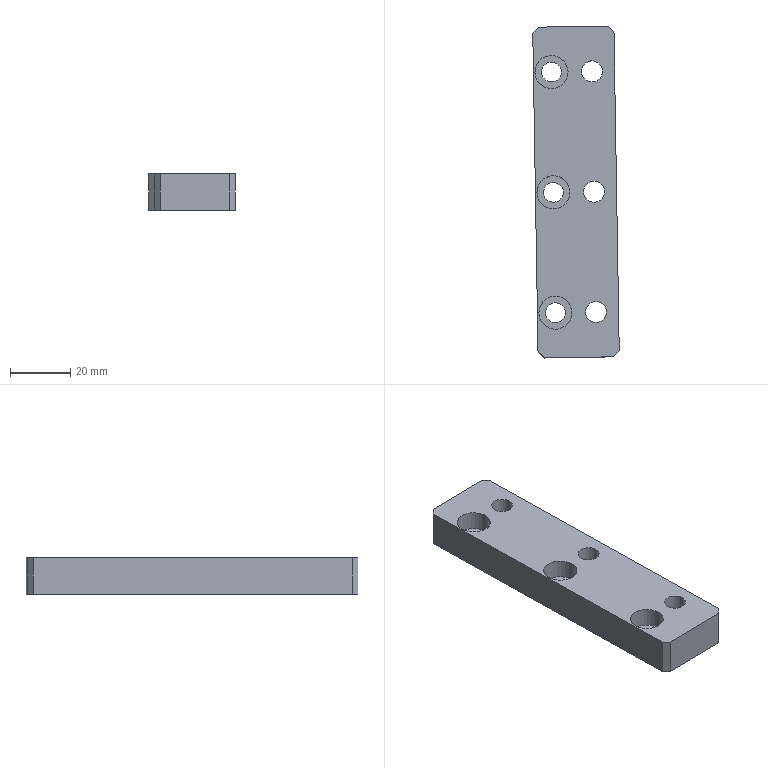Component | SolidWorks | 8TC-A17001-20-09MountingPlate1-2 | 1 solid | 31 faces | box 28.74 x 110.36 x 12 mm | volume 31759 mm3 | cylinder 18 | plane 13 | commonest cylinder face diameters 11 x6 6.6 x6 7 x6 | material A3
build123d program:
from build123d import *

# Parameters (mm, degrees)
SKETCH1_W                                       = 110
SKETCH1_H                                       = 27
BOSS_EXTRUDE1_DEPTH                             = 12
SKETCH2_R                                       = 3.5
CUT_EXTRUDE1_DEPTH                              = 58.89
M6_HEX_SOCKET_HEAD_CAP_SCREW_CBORE1_D           = 6.6
M6_HEX_SOCKET_HEAD_CAP_SCREW_CBORE1_CBORE_D     = 11
M6_HEX_SOCKET_HEAD_CAP_SCREW_CBORE1_CBORE_DEPTH = 6.4
CHAMFER1_SIZE                                   = 2


with BuildPart() as part:
    # Sketch1 → Boss-Extrude1 (new body)
    with BuildSketch(Plane(origin=(0, 0, 0), x_dir=(1, 0, 0), z_dir=(0, 1, 0))):
        Rectangle(SKETCH1_W, SKETCH1_H)
    extrude(amount=BOSS_EXTRUDE1_DEPTH)

    # Sketch2 → Cut-Extrude1 (cut, through all)
    with BuildSketch(Plane(origin=(0, 12, 0), x_dir=(1, 0, 0), z_dir=(0, 1, 0))):
        with Locations(Location((-40, -6, 0), (0, 0, 270))):
            Circle(SKETCH2_R)
        with Locations(Location((0, -6, 0), (0, 0, 270))):
            Circle(SKETCH2_R)
        with Locations(Location((40, -6, 0), (0, 0, 90))):
            Circle(SKETCH2_R)
    extrude(amount=-CUT_EXTRUDE1_DEPTH, mode=Mode.SUBTRACT)

    # M6 Hex Socket Head Cap Screw CBORE1 (through all)
    with Locations(Plane(origin=(0, 0, 0), x_dir=(-1, 0, 0), z_dir=(0, -1, 0))):
        with Locations((40, 7.5), (0, 7.5), (-40, 7.5)):
            CounterBoreHole(M6_HEX_SOCKET_HEAD_CAP_SCREW_CBORE1_D / 2, M6_HEX_SOCKET_HEAD_CAP_SCREW_CBORE1_CBORE_D / 2, M6_HEX_SOCKET_HEAD_CAP_SCREW_CBORE1_CBORE_DEPTH)

    # Chamfer1
    chamfer1_edges = [part.edges().sort_by_distance(p)[0] for p in [
        (55, 6, 13.5),
        (-55, 6, 13.5),
        (-55, 6, -13.5),
        (55, 6, -13.5),
    ]]
    chamfer(chamfer1_edges, length=CHAMFER1_SIZE)


solid = part.part

# Placed as in the assembly
solid = solid.moved(Location((802.019, 201.857, 42.5), (-90, 89.057, 0)))
STEP:
#1=COLOUR_RGB('',0.7922,0.8196,0.9333);
#2=FILL_AREA_STYLE_COLOUR('',#1);
#3=FILL_AREA_STYLE('',(#2));
#4=SURFACE_STYLE_FILL_AREA(#3);
#5=SURFACE_SIDE_STYLE('',(#4));
#6=SURFACE_STYLE_USAGE(.BOTH.,#5);
#7=PRESENTATION_STYLE_ASSIGNMENT((#6));
#8=CARTESIAN_POINT('',(31.471,9.52,1.421));
#9=VERTEX_POINT('',#8);
#10=CARTESIAN_POINT('',(31.038,9.513,1.421));
#11=VERTEX_POINT('',#10);
#12=CARTESIAN_POINT('',(31.254,9.517,1.421));
#13=DIRECTION('',(0.,-0.,1.));
#14=DIRECTION('',(-0.9999,-0.01645,0.));
#15=AXIS2_PLACEMENT_3D('',#12,#13,#14);
#16=CIRCLE('',#15,0.2165);
#17=EDGE_CURVE('',#9,#11,#16,.T.);
#18=ORIENTED_EDGE('',*,*,#17,.F.);
#19=CARTESIAN_POINT('',(31.471,9.52,1.673));
#20=VERTEX_POINT('',#19);
#21=CARTESIAN_POINT('',(31.471,9.52,1.673));
#22=DIRECTION('',(0.,-0.,1.));
#23=VECTOR('',#22,39.37);
#24=LINE('',#21,#23);
#25=EDGE_CURVE('',#9,#20,#24,.T.);
#26=ORIENTED_EDGE('',*,*,#25,.T.);
#27=CARTESIAN_POINT('',(31.038,9.513,1.673));
#28=VERTEX_POINT('',#27);
#29=CARTESIAN_POINT('',(31.254,9.517,1.673));
#30=DIRECTION('',(0.,-0.,1.));
#31=DIRECTION('',(-0.9999,-0.01645,0.));
#32=AXIS2_PLACEMENT_3D('',#29,#30,#31);
#33=CIRCLE('',#32,0.2165);
#34=EDGE_CURVE('',#20,#28,#33,.T.);
#35=ORIENTED_EDGE('',*,*,#34,.T.);
#36=CARTESIAN_POINT('',(31.038,9.513,1.673));
#37=DIRECTION('',(0.,-0.,1.));
#38=VECTOR('',#37,39.37);
#39=LINE('',#36,#38);
#40=EDGE_CURVE('',#11,#28,#39,.T.);
#41=ORIENTED_EDGE('',*,*,#40,.F.);
#42=EDGE_LOOP('',(#18,#26,#35,#41));
#43=FACE_OUTER_BOUND('',#42,.T.);
#44=CARTESIAN_POINT('',(31.254,9.517,1.673));
#45=DIRECTION('',(0.,-0.,1.));
#46=DIRECTION('',(-0.9999,-0.01645,0.));
#47=AXIS2_PLACEMENT_3D('',#44,#45,#46);
#48=CYLINDRICAL_SURFACE('',#47,0.2165);
#49=ADVANCED_FACE('',(#43),#48,.F.);
#50=CARTESIAN_POINT('',(31.384,9.519,1.201));
#51=VERTEX_POINT('',#50);
#52=CARTESIAN_POINT('',(31.125,9.515,1.201));
#53=VERTEX_POINT('',#52);
#54=CARTESIAN_POINT('',(31.254,9.517,1.201));
#55=DIRECTION('',(0.,-0.,1.));
#56=DIRECTION('',(-0.9999,-0.01645,0.));
#57=AXIS2_PLACEMENT_3D('',#54,#55,#56);
#58=CIRCLE('',#57,0.1299);
#59=EDGE_CURVE('',#51,#53,#58,.T.);
#60=ORIENTED_EDGE('',*,*,#59,.F.);
#61=CARTESIAN_POINT('',(31.384,9.519,1.421));
#62=VERTEX_POINT('',#61);
#63=CARTESIAN_POINT('',(31.384,9.519,1.673));
#64=DIRECTION('',(0.,-0.,1.));
#65=VECTOR('',#64,39.37);
#66=LINE('',#63,#65);
#67=EDGE_CURVE('',#51,#62,#66,.T.);
#68=ORIENTED_EDGE('',*,*,#67,.T.);
#69=CARTESIAN_POINT('',(31.125,9.515,1.421));
#70=VERTEX_POINT('',#69);
#71=CARTESIAN_POINT('',(31.254,9.517,1.421));
#72=DIRECTION('',(0.,-0.,1.));
#73=DIRECTION('',(-0.9999,-0.01645,0.));
#74=AXIS2_PLACEMENT_3D('',#71,#72,#73);
#75=CIRCLE('',#74,0.1299);
#76=EDGE_CURVE('',#62,#70,#75,.T.);
#77=ORIENTED_EDGE('',*,*,#76,.T.);
#78=CARTESIAN_POINT('',(31.125,9.515,1.673));
#79=DIRECTION('',(0.,-0.,1.));
#80=VECTOR('',#79,39.37);
#81=LINE('',#78,#80);
#82=EDGE_CURVE('',#53,#70,#81,.T.);
#83=ORIENTED_EDGE('',*,*,#82,.F.);
#84=EDGE_LOOP('',(#60,#68,#77,#83));
#85=FACE_OUTER_BOUND('',#84,.T.);
#86=CARTESIAN_POINT('',(31.254,9.517,1.673));
#87=DIRECTION('',(0.,-0.,1.));
#88=DIRECTION('',(-0.9999,-0.01645,0.));
#89=AXIS2_PLACEMENT_3D('',#86,#87,#88);
#90=CYLINDRICAL_SURFACE('',#89,0.1299);
#91=ADVANCED_FACE('',(#85),#90,.F.);
#92=CARTESIAN_POINT('',(31.497,7.946,1.421));
#93=VERTEX_POINT('',#92);
#94=CARTESIAN_POINT('',(31.064,7.939,1.421));
#95=VERTEX_POINT('',#94);
#96=CARTESIAN_POINT('',(31.28,7.942,1.421));
#97=DIRECTION('',(0.,-0.,1.));
#98=DIRECTION('',(-0.9999,-0.01645,0.));
#99=AXIS2_PLACEMENT_3D('',#96,#97,#98);
#100=CIRCLE('',#99,0.2165);
#101=EDGE_CURVE('',#93,#95,#100,.T.);
#102=ORIENTED_EDGE('',*,*,#101,.F.);
#103=CARTESIAN_POINT('',(31.497,7.946,1.673));
#104=VERTEX_POINT('',#103);
#105=CARTESIAN_POINT('',(31.497,7.946,1.673));
#106=DIRECTION('',(0.,-0.,1.));
#107=VECTOR('',#106,39.37);
#108=LINE('',#105,#107);
#109=EDGE_CURVE('',#93,#104,#108,.T.);
#110=ORIENTED_EDGE('',*,*,#109,.T.);
#111=CARTESIAN_POINT('',(31.064,7.939,1.673));
#112=VERTEX_POINT('',#111);
#113=CARTESIAN_POINT('',(31.28,7.942,1.673));
#114=DIRECTION('',(0.,-0.,1.));
#115=DIRECTION('',(-0.9999,-0.01645,0.));
#116=AXIS2_PLACEMENT_3D('',#113,#114,#115);
#117=CIRCLE('',#116,0.2165);
#118=EDGE_CURVE('',#104,#112,#117,.T.);
#119=ORIENTED_EDGE('',*,*,#118,.T.);
#120=CARTESIAN_POINT('',(31.064,7.939,1.673));
#121=DIRECTION('',(0.,-0.,1.));
#122=VECTOR('',#121,39.37);
#123=LINE('',#120,#122);
#124=EDGE_CURVE('',#95,#112,#123,.T.);
#125=ORIENTED_EDGE('',*,*,#124,.F.);
#126=EDGE_LOOP('',(#102,#110,#119,#125));
#127=FACE_OUTER_BOUND('',#126,.T.);
#128=CARTESIAN_POINT('',(31.28,7.942,1.673));
#129=DIRECTION('',(0.,-0.,1.));
#130=DIRECTION('',(-0.9999,-0.01645,0.));
#131=AXIS2_PLACEMENT_3D('',#128,#129,#130);
#132=CYLINDRICAL_SURFACE('',#131,0.2165);
#133=ADVANCED_FACE('',(#127),#132,.F.);
#134=CARTESIAN_POINT('',(31.41,7.944,1.201));
#135=VERTEX_POINT('',#134);
#136=CARTESIAN_POINT('',(31.15,7.94,1.201));
#137=VERTEX_POINT('',#136);
#138=CARTESIAN_POINT('',(31.28,7.942,1.201));
#139=DIRECTION('',(0.,-0.,1.));
#140=DIRECTION('',(-0.9999,-0.01645,0.));
#141=AXIS2_PLACEMENT_3D('',#138,#139,#140);
#142=CIRCLE('',#141,0.1299);
#143=EDGE_CURVE('',#135,#137,#142,.T.);
#144=ORIENTED_EDGE('',*,*,#143,.F.);
#145=CARTESIAN_POINT('',(31.41,7.944,1.421));
#146=VERTEX_POINT('',#145);
#147=CARTESIAN_POINT('',(31.41,7.944,1.673));
#148=DIRECTION('',(0.,-0.,1.));
#149=VECTOR('',#148,39.37);
#150=LINE('',#147,#149);
#151=EDGE_CURVE('',#135,#146,#150,.T.);
#152=ORIENTED_EDGE('',*,*,#151,.T.);
#153=CARTESIAN_POINT('',(31.15,7.94,1.421));
#154=VERTEX_POINT('',#153);
#155=CARTESIAN_POINT('',(31.28,7.942,1.421));
#156=DIRECTION('',(0.,-0.,1.));
#157=DIRECTION('',(-0.9999,-0.01645,0.));
#158=AXIS2_PLACEMENT_3D('',#155,#156,#157);
#159=CIRCLE('',#158,0.1299);
#160=EDGE_CURVE('',#146,#154,#159,.T.);
#161=ORIENTED_EDGE('',*,*,#160,.T.);
#162=CARTESIAN_POINT('',(31.15,7.94,1.673));
#163=DIRECTION('',(0.,-0.,1.));
#164=VECTOR('',#163,39.37);
#165=LINE('',#162,#164);
#166=EDGE_CURVE('',#137,#154,#165,.T.);
#167=ORIENTED_EDGE('',*,*,#166,.F.);
#168=EDGE_LOOP('',(#144,#152,#161,#167));
#169=FACE_OUTER_BOUND('',#168,.T.);
#170=CARTESIAN_POINT('',(31.28,7.942,1.673));
#171=DIRECTION('',(0.,-0.,1.));
#172=DIRECTION('',(-0.9999,-0.01645,0.));
#173=AXIS2_PLACEMENT_3D('',#170,#171,#172);
#174=CYLINDRICAL_SURFACE('',#173,0.1299);
#175=ADVANCED_FACE('',(#169),#174,.F.);
#176=CARTESIAN_POINT('',(31.523,6.371,1.421));
#177=VERTEX_POINT('',#176);
#178=CARTESIAN_POINT('',(31.09,6.364,1.421));
#179=VERTEX_POINT('',#178);
#180=CARTESIAN_POINT('',(31.306,6.368,1.421));
#181=DIRECTION('',(0.,-0.,1.));
#182=DIRECTION('',(-0.9999,-0.01645,0.));
#183=AXIS2_PLACEMENT_3D('',#180,#181,#182);
#184=CIRCLE('',#183,0.2165);
#185=EDGE_CURVE('',#177,#179,#184,.T.);
#186=ORIENTED_EDGE('',*,*,#185,.F.);
#187=CARTESIAN_POINT('',(31.523,6.371,1.673));
#188=VERTEX_POINT('',#187);
#189=CARTESIAN_POINT('',(31.523,6.371,1.673));
#190=DIRECTION('',(0.,-0.,1.));
#191=VECTOR('',#190,39.37);
#192=LINE('',#189,#191);
#193=EDGE_CURVE('',#177,#188,#192,.T.);
#194=ORIENTED_EDGE('',*,*,#193,.T.);
#195=CARTESIAN_POINT('',(31.09,6.364,1.673));
#196=VERTEX_POINT('',#195);
#197=CARTESIAN_POINT('',(31.306,6.368,1.673));
#198=DIRECTION('',(0.,-0.,1.));
#199=DIRECTION('',(-0.9999,-0.01645,0.));
#200=AXIS2_PLACEMENT_3D('',#197,#198,#199);
#201=CIRCLE('',#200,0.2165);
#202=EDGE_CURVE('',#188,#196,#201,.T.);
#203=ORIENTED_EDGE('',*,*,#202,.T.);
#204=CARTESIAN_POINT('',(31.09,6.364,1.673));
#205=DIRECTION('',(0.,-0.,1.));
#206=VECTOR('',#205,39.37);
#207=LINE('',#204,#206);
#208=EDGE_CURVE('',#179,#196,#207,.T.);
#209=ORIENTED_EDGE('',*,*,#208,.F.);
#210=EDGE_LOOP('',(#186,#194,#203,#209));
#211=FACE_OUTER_BOUND('',#210,.T.);
#212=CARTESIAN_POINT('',(31.306,6.368,1.673));
#213=DIRECTION('',(0.,-0.,1.));
#214=DIRECTION('',(-0.9999,-0.01645,0.));
#215=AXIS2_PLACEMENT_3D('',#212,#213,#214);
#216=CYLINDRICAL_SURFACE('',#215,0.2165);
#217=ADVANCED_FACE('',(#211),#216,.F.);
#218=CARTESIAN_POINT('',(31.436,6.37,1.201));
#219=VERTEX_POINT('',#218);
#220=CARTESIAN_POINT('',(31.176,6.366,1.201));
#221=VERTEX_POINT('',#220);
#222=CARTESIAN_POINT('',(31.306,6.368,1.201));
#223=DIRECTION('',(0.,-0.,1.));
#224=DIRECTION('',(-0.9999,-0.01645,0.));
#225=AXIS2_PLACEMENT_3D('',#222,#223,#224);
#226=CIRCLE('',#225,0.1299);
#227=EDGE_CURVE('',#219,#221,#226,.T.);
#228=ORIENTED_EDGE('',*,*,#227,.F.);
#229=CARTESIAN_POINT('',(31.436,6.37,1.421));
#230=VERTEX_POINT('',#229);
#231=CARTESIAN_POINT('',(31.436,6.37,1.673));
#232=DIRECTION('',(0.,-0.,1.));
#233=VECTOR('',#232,39.37);
#234=LINE('',#231,#233);
#235=EDGE_CURVE('',#219,#230,#234,.T.);
#236=ORIENTED_EDGE('',*,*,#235,.T.);
#237=CARTESIAN_POINT('',(31.176,6.366,1.421));
#238=VERTEX_POINT('',#237);
#239=CARTESIAN_POINT('',(31.306,6.368,1.421));
#240=DIRECTION('',(0.,-0.,1.));
#241=DIRECTION('',(-0.9999,-0.01645,0.));
#242=AXIS2_PLACEMENT_3D('',#239,#240,#241);
#243=CIRCLE('',#242,0.1299);
#244=EDGE_CURVE('',#230,#238,#243,.T.);
#245=ORIENTED_EDGE('',*,*,#244,.T.);
#246=CARTESIAN_POINT('',(31.176,6.366,1.673));
#247=DIRECTION('',(0.,-0.,1.));
#248=VECTOR('',#247,39.37);
#249=LINE('',#246,#248);
#250=EDGE_CURVE('',#221,#238,#249,.T.);
#251=ORIENTED_EDGE('',*,*,#250,.F.);
#252=EDGE_LOOP('',(#228,#236,#245,#251));
#253=FACE_OUTER_BOUND('',#252,.T.);
#254=CARTESIAN_POINT('',(31.306,6.368,1.673));
#255=DIRECTION('',(0.,-0.,1.));
#256=DIRECTION('',(-0.9999,-0.01645,0.));
#257=AXIS2_PLACEMENT_3D('',#254,#255,#256);
#258=CYLINDRICAL_SURFACE('',#257,0.1299);
#259=ADVANCED_FACE('',(#253),#258,.F.);
#260=CARTESIAN_POINT('',(31.7,6.374,1.673));
#261=VERTEX_POINT('',#260);
#262=CARTESIAN_POINT('',(31.975,6.379,1.673));
#263=VERTEX_POINT('',#262);
#264=CARTESIAN_POINT('',(31.838,6.376,1.673));
#265=DIRECTION('',(-0.,0.,-1.));
#266=DIRECTION('',(-0.9999,-0.01645,0.));
#267=AXIS2_PLACEMENT_3D('',#264,#265,#266);
#268=CIRCLE('',#267,0.1378);
#269=EDGE_CURVE('',#261,#263,#268,.T.);
#270=ORIENTED_EDGE('',*,*,#269,.F.);
#271=CARTESIAN_POINT('',(31.7,6.374,1.201));
#272=VERTEX_POINT('',#271);
#273=CARTESIAN_POINT('',(31.7,6.374,1.673));
#274=DIRECTION('',(-0.,0.,-1.));
#275=VECTOR('',#274,39.37);
#276=LINE('',#273,#275);
#277=EDGE_CURVE('',#261,#272,#276,.T.);
#278=ORIENTED_EDGE('',*,*,#277,.T.);
#279=CARTESIAN_POINT('',(31.975,6.379,1.201));
#280=VERTEX_POINT('',#279);
#281=CARTESIAN_POINT('',(31.838,6.376,1.201));
#282=DIRECTION('',(-0.,0.,-1.));
#283=DIRECTION('',(-0.9999,-0.01645,0.));
#284=AXIS2_PLACEMENT_3D('',#281,#282,#283);
#285=CIRCLE('',#284,0.1378);
#286=EDGE_CURVE('',#272,#280,#285,.T.);
#287=ORIENTED_EDGE('',*,*,#286,.T.);
#288=CARTESIAN_POINT('',(31.975,6.379,1.673));
#289=DIRECTION('',(-0.,0.,-1.));
#290=VECTOR('',#289,39.37);
#291=LINE('',#288,#290);
#292=EDGE_CURVE('',#263,#280,#291,.T.);
#293=ORIENTED_EDGE('',*,*,#292,.F.);
#294=EDGE_LOOP('',(#270,#278,#287,#293));
#295=FACE_OUTER_BOUND('',#294,.T.);
#296=CARTESIAN_POINT('',(31.838,6.376,1.673));
#297=DIRECTION('',(-0.,0.,-1.));
#298=DIRECTION('',(0.9999,0.01645,0.));
#299=AXIS2_PLACEMENT_3D('',#296,#297,#298);
#300=CYLINDRICAL_SURFACE('',#299,0.1378);
#301=ADVANCED_FACE('',(#295),#300,.F.);
#302=CARTESIAN_POINT('',(31.674,7.949,1.673));
#303=VERTEX_POINT('',#302);
#304=CARTESIAN_POINT('',(31.95,7.953,1.673));
#305=VERTEX_POINT('',#304);
#306=CARTESIAN_POINT('',(31.812,7.951,1.673));
#307=DIRECTION('',(-0.,0.,-1.));
#308=DIRECTION('',(0.9999,0.01645,0.));
#309=AXIS2_PLACEMENT_3D('',#306,#307,#308);
#310=CIRCLE('',#309,0.1378);
#311=EDGE_CURVE('',#303,#305,#310,.T.);
#312=ORIENTED_EDGE('',*,*,#311,.F.);
#313=CARTESIAN_POINT('',(31.674,7.949,1.201));
#314=VERTEX_POINT('',#313);
#315=CARTESIAN_POINT('',(31.674,7.949,1.673));
#316=DIRECTION('',(-0.,0.,-1.));
#317=VECTOR('',#316,39.37);
#318=LINE('',#315,#317);
#319=EDGE_CURVE('',#303,#314,#318,.T.);
#320=ORIENTED_EDGE('',*,*,#319,.T.);
#321=CARTESIAN_POINT('',(31.95,7.953,1.201));
#322=VERTEX_POINT('',#321);
#323=CARTESIAN_POINT('',(31.812,7.951,1.201));
#324=DIRECTION('',(-0.,0.,-1.));
#325=DIRECTION('',(0.9999,0.01645,0.));
#326=AXIS2_PLACEMENT_3D('',#323,#324,#325);
#327=CIRCLE('',#326,0.1378);
#328=EDGE_CURVE('',#314,#322,#327,.T.);
#329=ORIENTED_EDGE('',*,*,#328,.T.);
#330=CARTESIAN_POINT('',(31.95,7.953,1.673));
#331=DIRECTION('',(-0.,0.,-1.));
#332=VECTOR('',#331,39.37);
#333=LINE('',#330,#332);
#334=EDGE_CURVE('',#305,#322,#333,.T.);
#335=ORIENTED_EDGE('',*,*,#334,.F.);
#336=EDGE_LOOP('',(#312,#320,#329,#335));
#337=FACE_OUTER_BOUND('',#336,.T.);
#338=CARTESIAN_POINT('',(31.812,7.951,1.673));
#339=DIRECTION('',(-0.,0.,-1.));
#340=DIRECTION('',(0.9999,0.01645,0.));
#341=AXIS2_PLACEMENT_3D('',#338,#339,#340);
#342=CYLINDRICAL_SURFACE('',#341,0.1378);
#343=ADVANCED_FACE('',(#337),#342,.F.);
#344=CARTESIAN_POINT('',(31.648,9.523,1.673));
#345=VERTEX_POINT('',#344);
#346=CARTESIAN_POINT('',(31.924,9.528,1.673));
#347=VERTEX_POINT('',#346);
#348=CARTESIAN_POINT('',(31.786,9.526,1.673));
#349=DIRECTION('',(-0.,0.,-1.));
#350=DIRECTION('',(0.9999,0.01645,0.));
#351=AXIS2_PLACEMENT_3D('',#348,#349,#350);
#352=CIRCLE('',#351,0.1378);
#353=EDGE_CURVE('',#345,#347,#352,.T.);
#354=ORIENTED_EDGE('',*,*,#353,.F.);
#355=CARTESIAN_POINT('',(31.648,9.523,1.201));
#356=VERTEX_POINT('',#355);
#357=CARTESIAN_POINT('',(31.648,9.523,1.673));
#358=DIRECTION('',(-0.,0.,-1.));
#359=VECTOR('',#358,39.37);
#360=LINE('',#357,#359);
#361=EDGE_CURVE('',#345,#356,#360,.T.);
#362=ORIENTED_EDGE('',*,*,#361,.T.);
#363=CARTESIAN_POINT('',(31.924,9.528,1.201));
#364=VERTEX_POINT('',#363);
#365=CARTESIAN_POINT('',(31.786,9.526,1.201));
#366=DIRECTION('',(-0.,0.,-1.));
#367=DIRECTION('',(0.9999,0.01645,0.));
#368=AXIS2_PLACEMENT_3D('',#365,#366,#367);
#369=CIRCLE('',#368,0.1378);
#370=EDGE_CURVE('',#356,#364,#369,.T.);
#371=ORIENTED_EDGE('',*,*,#370,.T.);
#372=CARTESIAN_POINT('',(31.924,9.528,1.673));
#373=DIRECTION('',(-0.,0.,-1.));
#374=VECTOR('',#373,39.37);
#375=LINE('',#372,#374);
#376=EDGE_CURVE('',#347,#364,#375,.T.);
#377=ORIENTED_EDGE('',*,*,#376,.F.);
#378=EDGE_LOOP('',(#354,#362,#371,#377));
#379=FACE_OUTER_BOUND('',#378,.T.);
#380=CARTESIAN_POINT('',(31.786,9.526,1.673));
#381=DIRECTION('',(-0.,0.,-1.));
#382=DIRECTION('',(0.9999,0.01645,0.));
#383=AXIS2_PLACEMENT_3D('',#380,#381,#382);
#384=CYLINDRICAL_SURFACE('',#383,0.1378);
#385=ADVANCED_FACE('',(#379),#384,.F.);
#386=CARTESIAN_POINT('',(32.064,5.79,1.673));
#387=VERTEX_POINT('',#386);
#388=CARTESIAN_POINT('',(31.158,5.775,1.673));
#389=VERTEX_POINT('',#388);
#390=CARTESIAN_POINT('',(31.08,5.773,1.673));
#391=DIRECTION('',(-0.9999,-0.01645,0.));
#392=VECTOR('',#391,39.37);
#393=LINE('',#390,#392);
#394=EDGE_CURVE('',#387,#389,#393,.T.);
#395=ORIENTED_EDGE('',*,*,#394,.T.);
#396=CARTESIAN_POINT('',(31.158,5.775,1.201));
#397=VERTEX_POINT('',#396);
#398=CARTESIAN_POINT('',(31.158,5.775,1.201));
#399=DIRECTION('',(-0.,0.,-1.));
#400=VECTOR('',#399,39.37);
#401=LINE('',#398,#400);
#402=EDGE_CURVE('',#389,#397,#401,.T.);
#403=ORIENTED_EDGE('',*,*,#402,.T.);
#404=CARTESIAN_POINT('',(32.064,5.79,1.201));
#405=VERTEX_POINT('',#404);
#406=CARTESIAN_POINT('',(31.08,5.773,1.201));
#407=DIRECTION('',(-0.9999,-0.01645,0.));
#408=VECTOR('',#407,39.37);
#409=LINE('',#406,#408);
#410=EDGE_CURVE('',#405,#397,#409,.T.);
#411=ORIENTED_EDGE('',*,*,#410,.F.);
#412=CARTESIAN_POINT('',(32.064,5.79,1.201));
#413=DIRECTION('',(0.,-0.,1.));
#414=VECTOR('',#413,39.37);
#415=LINE('',#412,#414);
#416=EDGE_CURVE('',#405,#387,#415,.T.);
#417=ORIENTED_EDGE('',*,*,#416,.T.);
#418=EDGE_LOOP('',(#395,#403,#411,#417));
#419=FACE_OUTER_BOUND('',#418,.T.);
#420=CARTESIAN_POINT('',(31.08,5.773,1.201));
#421=DIRECTION('',(-0.01645,0.9999,0.));
#422=DIRECTION('',(0.9999,0.01645,-0.));
#423=AXIS2_PLACEMENT_3D('',#420,#421,#422);
#424=PLANE('',#423);
#425=ADVANCED_FACE('',(#419),#424,.F.);
#426=CARTESIAN_POINT('',(31.078,5.852,1.673));
#427=VERTEX_POINT('',#426);
#428=CARTESIAN_POINT('',(31.01,10.025,1.673));
#429=VERTEX_POINT('',#428);
#430=CARTESIAN_POINT('',(31.009,10.103,1.673));
#431=DIRECTION('',(-0.01645,0.9999,0.));
#432=VECTOR('',#431,39.37);
#433=LINE('',#430,#432);
#434=EDGE_CURVE('',#427,#429,#433,.T.);
#435=ORIENTED_EDGE('',*,*,#434,.T.);
#436=CARTESIAN_POINT('',(31.01,10.025,1.201));
#437=VERTEX_POINT('',#436);
#438=CARTESIAN_POINT('',(31.01,10.025,1.201));
#439=DIRECTION('',(-0.,0.,-1.));
#440=VECTOR('',#439,39.37);
#441=LINE('',#438,#440);
#442=EDGE_CURVE('',#429,#437,#441,.T.);
#443=ORIENTED_EDGE('',*,*,#442,.T.);
#444=CARTESIAN_POINT('',(31.078,5.852,1.201));
#445=VERTEX_POINT('',#444);
#446=CARTESIAN_POINT('',(31.009,10.103,1.201));
#447=DIRECTION('',(-0.01645,0.9999,0.));
#448=VECTOR('',#447,39.37);
#449=LINE('',#446,#448);
#450=EDGE_CURVE('',#445,#437,#449,.T.);
#451=ORIENTED_EDGE('',*,*,#450,.F.);
#452=CARTESIAN_POINT('',(31.078,5.852,1.201));
#453=DIRECTION('',(0.,-0.,1.));
#454=VECTOR('',#453,39.37);
#455=LINE('',#452,#454);
#456=EDGE_CURVE('',#445,#427,#455,.T.);
#457=ORIENTED_EDGE('',*,*,#456,.T.);
#458=EDGE_LOOP('',(#435,#443,#451,#457));
#459=FACE_OUTER_BOUND('',#458,.T.);
#460=CARTESIAN_POINT('',(31.009,10.103,1.201));
#461=DIRECTION('',(0.9999,0.01645,-0.));
#462=DIRECTION('',(0.01645,-0.9999,-0.));
#463=AXIS2_PLACEMENT_3D('',#460,#461,#462);
#464=PLANE('',#463);
#465=ADVANCED_FACE('',(#459),#464,.F.);
#466=CARTESIAN_POINT('',(31.087,10.105,1.201));
#467=VERTEX_POINT('',#466);
#468=CARTESIAN_POINT('',(31.993,10.12,1.201));
#469=VERTEX_POINT('',#468);
#470=CARTESIAN_POINT('',(31.009,10.103,1.201));
#471=DIRECTION('',(0.9999,0.01645,-0.));
#472=VECTOR('',#471,39.37);
#473=LINE('',#470,#472);
#474=EDGE_CURVE('',#467,#469,#473,.T.);
#475=ORIENTED_EDGE('',*,*,#474,.F.);
#476=CARTESIAN_POINT('',(31.087,10.105,1.673));
#477=VERTEX_POINT('',#476);
#478=CARTESIAN_POINT('',(31.087,10.105,1.201));
#479=DIRECTION('',(0.,-0.,1.));
#480=VECTOR('',#479,39.37);
#481=LINE('',#478,#480);
#482=EDGE_CURVE('',#467,#477,#481,.T.);
#483=ORIENTED_EDGE('',*,*,#482,.T.);
#484=CARTESIAN_POINT('',(31.993,10.12,1.673));
#485=VERTEX_POINT('',#484);
#486=CARTESIAN_POINT('',(31.009,10.103,1.673));
#487=DIRECTION('',(0.9999,0.01645,-0.));
#488=VECTOR('',#487,39.37);
#489=LINE('',#486,#488);
#490=EDGE_CURVE('',#477,#485,#489,.T.);
#491=ORIENTED_EDGE('',*,*,#490,.T.);
#492=CARTESIAN_POINT('',(31.993,10.12,1.201));
#493=DIRECTION('',(-0.,0.,-1.));
#494=VECTOR('',#493,39.37);
#495=LINE('',#492,#494);
#496=EDGE_CURVE('',#485,#469,#495,.T.);
#497=ORIENTED_EDGE('',*,*,#496,.T.);
#498=EDGE_LOOP('',(#475,#483,#491,#497));
#499=FACE_OUTER_BOUND('',#498,.T.);
#500=CARTESIAN_POINT('',(31.009,10.103,1.201));
#501=DIRECTION('',(0.01645,-0.9999,-0.));
#502=DIRECTION('',(-0.9999,-0.01645,0.));
#503=AXIS2_PLACEMENT_3D('',#500,#501,#502);
#504=PLANE('',#503);
#505=ADVANCED_FACE('',(#499),#504,.F.);
#506=CARTESIAN_POINT('',(32.073,10.042,1.673));
#507=VERTEX_POINT('',#506);
#508=CARTESIAN_POINT('',(32.141,5.87,1.673));
#509=VERTEX_POINT('',#508);
#510=CARTESIAN_POINT('',(32.071,10.121,1.673));
#511=DIRECTION('',(0.01645,-0.9999,-0.));
#512=VECTOR('',#511,39.37);
#513=LINE('',#510,#512);
#514=EDGE_CURVE('',#507,#509,#513,.T.);
#515=ORIENTED_EDGE('',*,*,#514,.T.);
#516=CARTESIAN_POINT('',(32.141,5.87,1.201));
#517=VERTEX_POINT('',#516);
#518=CARTESIAN_POINT('',(32.141,5.87,1.201));
#519=DIRECTION('',(-0.,0.,-1.));
#520=VECTOR('',#519,39.37);
#521=LINE('',#518,#520);
#522=EDGE_CURVE('',#509,#517,#521,.T.);
#523=ORIENTED_EDGE('',*,*,#522,.T.);
#524=CARTESIAN_POINT('',(32.073,10.042,1.201));
#525=VERTEX_POINT('',#524);
#526=CARTESIAN_POINT('',(32.071,10.121,1.201));
#527=DIRECTION('',(0.01645,-0.9999,-0.));
#528=VECTOR('',#527,39.37);
#529=LINE('',#526,#528);
#530=EDGE_CURVE('',#525,#517,#529,.T.);
#531=ORIENTED_EDGE('',*,*,#530,.F.);
#532=CARTESIAN_POINT('',(32.073,10.042,1.201));
#533=DIRECTION('',(0.,-0.,1.));
#534=VECTOR('',#533,39.37);
#535=LINE('',#532,#534);
#536=EDGE_CURVE('',#525,#507,#535,.T.);
#537=ORIENTED_EDGE('',*,*,#536,.T.);
#538=EDGE_LOOP('',(#515,#523,#531,#537));
#539=FACE_OUTER_BOUND('',#538,.T.);
#540=CARTESIAN_POINT('',(32.071,10.121,1.201));
#541=DIRECTION('',(-0.9999,-0.01645,0.));
#542=DIRECTION('',(-0.01645,0.9999,0.));
#543=AXIS2_PLACEMENT_3D('',#540,#541,#542);
#544=PLANE('',#543);
#545=ADVANCED_FACE('',(#539),#544,.F.);
#546=CARTESIAN_POINT('',(31.254,9.517,1.201));
#547=DIRECTION('',(0.,-0.,1.));
#548=DIRECTION('',(-0.9999,-0.01645,0.));
#549=AXIS2_PLACEMENT_3D('',#546,#547,#548);
#550=CIRCLE('',#549,0.1299);
#551=EDGE_CURVE('',#53,#51,#550,.T.);
#552=ORIENTED_EDGE('',*,*,#551,.T.);
#553=ORIENTED_EDGE('',*,*,#59,.T.);
#554=EDGE_LOOP('',(#552,#553));
#555=FACE_BOUND('',#554,.T.);
#556=CARTESIAN_POINT('',(31.28,7.942,1.201));
#557=DIRECTION('',(0.,-0.,1.));
#558=DIRECTION('',(-0.9999,-0.01645,0.));
#559=AXIS2_PLACEMENT_3D('',#556,#557,#558);
#560=CIRCLE('',#559,0.1299);
#561=EDGE_CURVE('',#137,#135,#560,.T.);
#562=ORIENTED_EDGE('',*,*,#561,.T.);
#563=ORIENTED_EDGE('',*,*,#143,.T.);
#564=EDGE_LOOP('',(#562,#563));
#565=FACE_BOUND('',#564,.T.);
#566=CARTESIAN_POINT('',(31.306,6.368,1.201));
#567=DIRECTION('',(0.,-0.,1.));
#568=DIRECTION('',(-0.9999,-0.01645,0.));
#569=AXIS2_PLACEMENT_3D('',#566,#567,#568);
#570=CIRCLE('',#569,0.1299);
#571=EDGE_CURVE('',#221,#219,#570,.T.);
#572=ORIENTED_EDGE('',*,*,#571,.T.);
#573=ORIENTED_EDGE('',*,*,#227,.T.);
#574=EDGE_LOOP('',(#572,#573));
#575=FACE_BOUND('',#574,.T.);
#576=CARTESIAN_POINT('',(31.838,6.376,1.201));
#577=DIRECTION('',(-0.,0.,-1.));
#578=DIRECTION('',(-0.9999,-0.01645,0.));
#579=AXIS2_PLACEMENT_3D('',#576,#577,#578);
#580=CIRCLE('',#579,0.1378);
#581=EDGE_CURVE('',#280,#272,#580,.T.);
#582=ORIENTED_EDGE('',*,*,#581,.F.);
#583=ORIENTED_EDGE('',*,*,#286,.F.);
#584=EDGE_LOOP('',(#582,#583));
#585=FACE_BOUND('',#584,.T.);
#586=CARTESIAN_POINT('',(31.812,7.951,1.201));
#587=DIRECTION('',(-0.,0.,-1.));
#588=DIRECTION('',(0.9999,0.01645,0.));
#589=AXIS2_PLACEMENT_3D('',#586,#587,#588);
#590=CIRCLE('',#589,0.1378);
#591=EDGE_CURVE('',#322,#314,#590,.T.);
#592=ORIENTED_EDGE('',*,*,#591,.F.);
#593=ORIENTED_EDGE('',*,*,#328,.F.);
#594=EDGE_LOOP('',(#592,#593));
#595=FACE_BOUND('',#594,.T.);
#596=CARTESIAN_POINT('',(31.786,9.526,1.201));
#597=DIRECTION('',(-0.,0.,-1.));
#598=DIRECTION('',(0.9999,0.01645,0.));
#599=AXIS2_PLACEMENT_3D('',#596,#597,#598);
#600=CIRCLE('',#599,0.1378);
#601=EDGE_CURVE('',#364,#356,#600,.T.);
#602=ORIENTED_EDGE('',*,*,#601,.F.);
#603=ORIENTED_EDGE('',*,*,#370,.F.);
#604=EDGE_LOOP('',(#602,#603));
#605=FACE_BOUND('',#604,.T.);
#606=ORIENTED_EDGE('',*,*,#450,.T.);
#607=CARTESIAN_POINT('',(30.245,9.234,1.201));
#608=DIRECTION('',(0.6954,0.7186,-0.));
#609=VECTOR('',#608,39.37);
#610=LINE('',#607,#609);
#611=EDGE_CURVE('',#437,#467,#610,.T.);
#612=ORIENTED_EDGE('',*,*,#611,.T.);
#613=ORIENTED_EDGE('',*,*,#474,.T.);
#614=CARTESIAN_POINT('',(32.863,9.278,1.201));
#615=DIRECTION('',(0.7186,-0.6954,-0.));
#616=VECTOR('',#615,39.37);
#617=LINE('',#614,#616);
#618=EDGE_CURVE('',#469,#525,#617,.T.);
#619=ORIENTED_EDGE('',*,*,#618,.T.);
#620=ORIENTED_EDGE('',*,*,#530,.T.);
#621=CARTESIAN_POINT('',(32.906,6.66,1.201));
#622=DIRECTION('',(-0.6954,-0.7186,0.));
#623=VECTOR('',#622,39.37);
#624=LINE('',#621,#623);
#625=EDGE_CURVE('',#517,#405,#624,.T.);
#626=ORIENTED_EDGE('',*,*,#625,.T.);
#627=ORIENTED_EDGE('',*,*,#410,.T.);
#628=CARTESIAN_POINT('',(30.288,6.617,1.201));
#629=DIRECTION('',(-0.7186,0.6954,0.));
#630=VECTOR('',#629,39.37);
#631=LINE('',#628,#630);
#632=EDGE_CURVE('',#397,#445,#631,.T.);
#633=ORIENTED_EDGE('',*,*,#632,.T.);
#634=EDGE_LOOP('',(#606,#612,#613,#619,#620,#626,#627,#633));
#635=FACE_OUTER_BOUND('',#634,.T.);
#636=CARTESIAN_POINT('',(31.576,7.947,1.201));
#637=DIRECTION('',(-0.,0.,-1.));
#638=DIRECTION('',(0.9999,0.01645,-0.));
#639=AXIS2_PLACEMENT_3D('',#636,#637,#638);
#640=PLANE('',#639);
#641=ADVANCED_FACE('',(#555,#565,#575,#585,#595,#605,#635),#640,.T.);
#642=CARTESIAN_POINT('',(31.254,9.517,1.673));
#643=DIRECTION('',(0.,-0.,1.));
#644=DIRECTION('',(-0.9999,-0.01645,0.));
#645=AXIS2_PLACEMENT_3D('',#642,#643,#644);
#646=CIRCLE('',#645,0.2165);
#647=EDGE_CURVE('',#28,#20,#646,.T.);
#648=ORIENTED_EDGE('',*,*,#647,.F.);
#649=ORIENTED_EDGE('',*,*,#34,.F.);
#650=EDGE_LOOP('',(#648,#649));
#651=FACE_BOUND('',#650,.T.);
#652=CARTESIAN_POINT('',(31.28,7.942,1.673));
#653=DIRECTION('',(0.,-0.,1.));
#654=DIRECTION('',(-0.9999,-0.01645,0.));
#655=AXIS2_PLACEMENT_3D('',#652,#653,#654);
#656=CIRCLE('',#655,0.2165);
#657=EDGE_CURVE('',#112,#104,#656,.T.);
#658=ORIENTED_EDGE('',*,*,#657,.F.);
#659=ORIENTED_EDGE('',*,*,#118,.F.);
#660=EDGE_LOOP('',(#658,#659));
#661=FACE_BOUND('',#660,.T.);
#662=CARTESIAN_POINT('',(31.306,6.368,1.673));
#663=DIRECTION('',(0.,-0.,1.));
#664=DIRECTION('',(-0.9999,-0.01645,0.));
#665=AXIS2_PLACEMENT_3D('',#662,#663,#664);
#666=CIRCLE('',#665,0.2165);
#667=EDGE_CURVE('',#196,#188,#666,.T.);
#668=ORIENTED_EDGE('',*,*,#667,.F.);
#669=ORIENTED_EDGE('',*,*,#202,.F.);
#670=EDGE_LOOP('',(#668,#669));
#671=FACE_BOUND('',#670,.T.);
#672=CARTESIAN_POINT('',(31.838,6.376,1.673));
#673=DIRECTION('',(-0.,0.,-1.));
#674=DIRECTION('',(-0.9999,-0.01645,0.));
#675=AXIS2_PLACEMENT_3D('',#672,#673,#674);
#676=CIRCLE('',#675,0.1378);
#677=EDGE_CURVE('',#263,#261,#676,.T.);
#678=ORIENTED_EDGE('',*,*,#677,.T.);
#679=ORIENTED_EDGE('',*,*,#269,.T.);
#680=EDGE_LOOP('',(#678,#679));
#681=FACE_BOUND('',#680,.T.);
#682=CARTESIAN_POINT('',(31.812,7.951,1.673));
#683=DIRECTION('',(-0.,0.,-1.));
#684=DIRECTION('',(0.9999,0.01645,0.));
#685=AXIS2_PLACEMENT_3D('',#682,#683,#684);
#686=CIRCLE('',#685,0.1378);
#687=EDGE_CURVE('',#305,#303,#686,.T.);
#688=ORIENTED_EDGE('',*,*,#687,.T.);
#689=ORIENTED_EDGE('',*,*,#311,.T.);
#690=EDGE_LOOP('',(#688,#689));
#691=FACE_BOUND('',#690,.T.);
#692=CARTESIAN_POINT('',(31.786,9.526,1.673));
#693=DIRECTION('',(-0.,0.,-1.));
#694=DIRECTION('',(0.9999,0.01645,0.));
#695=AXIS2_PLACEMENT_3D('',#692,#693,#694);
#696=CIRCLE('',#695,0.1378);
#697=EDGE_CURVE('',#347,#345,#696,.T.);
#698=ORIENTED_EDGE('',*,*,#697,.T.);
#699=ORIENTED_EDGE('',*,*,#353,.T.);
#700=EDGE_LOOP('',(#698,#699));
#701=FACE_BOUND('',#700,.T.);
#702=ORIENTED_EDGE('',*,*,#490,.F.);
#703=CARTESIAN_POINT('',(31.087,10.105,1.673));
#704=DIRECTION('',(-0.6954,-0.7186,0.));
#705=VECTOR('',#704,39.37);
#706=LINE('',#703,#705);
#707=EDGE_CURVE('',#477,#429,#706,.T.);
#708=ORIENTED_EDGE('',*,*,#707,.T.);
#709=ORIENTED_EDGE('',*,*,#434,.F.);
#710=CARTESIAN_POINT('',(31.078,5.852,1.673));
#711=DIRECTION('',(0.7186,-0.6954,-0.));
#712=VECTOR('',#711,39.37);
#713=LINE('',#710,#712);
#714=EDGE_CURVE('',#427,#389,#713,.T.);
#715=ORIENTED_EDGE('',*,*,#714,.T.);
#716=ORIENTED_EDGE('',*,*,#394,.F.);
#717=CARTESIAN_POINT('',(32.064,5.79,1.673));
#718=DIRECTION('',(0.6954,0.7186,-0.));
#719=VECTOR('',#718,39.37);
#720=LINE('',#717,#719);
#721=EDGE_CURVE('',#387,#509,#720,.T.);
#722=ORIENTED_EDGE('',*,*,#721,.T.);
#723=ORIENTED_EDGE('',*,*,#514,.F.);
#724=CARTESIAN_POINT('',(32.073,10.042,1.673));
#725=DIRECTION('',(-0.7186,0.6954,0.));
#726=VECTOR('',#725,39.37);
#727=LINE('',#724,#726);
#728=EDGE_CURVE('',#507,#485,#727,.T.);
#729=ORIENTED_EDGE('',*,*,#728,.T.);
#730=EDGE_LOOP('',(#702,#708,#709,#715,#716,#722,#723,#729));
#731=FACE_OUTER_BOUND('',#730,.T.);
#732=CARTESIAN_POINT('',(31.576,7.947,1.673));
#733=DIRECTION('',(-0.,0.,-1.));
#734=DIRECTION('',(0.9999,0.01645,-0.));
#735=AXIS2_PLACEMENT_3D('',#732,#733,#734);
#736=PLANE('',#735);
#737=ADVANCED_FACE('',(#651,#661,#671,#681,#691,#701,#731),#736,.F.);
#738=ORIENTED_EDGE('',*,*,#361,.F.);
#739=ORIENTED_EDGE('',*,*,#697,.F.);
#740=ORIENTED_EDGE('',*,*,#376,.T.);
#741=ORIENTED_EDGE('',*,*,#601,.T.);
#742=EDGE_LOOP('',(#738,#739,#740,#741));
#743=FACE_OUTER_BOUND('',#742,.T.);
#744=CARTESIAN_POINT('',(31.786,9.526,1.673));
#745=DIRECTION('',(-0.,0.,-1.));
#746=DIRECTION('',(0.9999,0.01645,0.));
#747=AXIS2_PLACEMENT_3D('',#744,#745,#746);
#748=CYLINDRICAL_SURFACE('',#747,0.1378);
#749=ADVANCED_FACE('',(#743),#748,.F.);
#750=ORIENTED_EDGE('',*,*,#319,.F.);
#751=ORIENTED_EDGE('',*,*,#687,.F.);
#752=ORIENTED_EDGE('',*,*,#334,.T.);
#753=ORIENTED_EDGE('',*,*,#591,.T.);
#754=EDGE_LOOP('',(#750,#751,#752,#753));
#755=FACE_OUTER_BOUND('',#754,.T.);
#756=CARTESIAN_POINT('',(31.812,7.951,1.673));
#757=DIRECTION('',(-0.,0.,-1.));
#758=DIRECTION('',(0.9999,0.01645,0.));
#759=AXIS2_PLACEMENT_3D('',#756,#757,#758);
#760=CYLINDRICAL_SURFACE('',#759,0.1378);
#761=ADVANCED_FACE('',(#755),#760,.F.);
#762=ORIENTED_EDGE('',*,*,#277,.F.);
#763=ORIENTED_EDGE('',*,*,#677,.F.);
#764=ORIENTED_EDGE('',*,*,#292,.T.);
#765=ORIENTED_EDGE('',*,*,#581,.T.);
#766=EDGE_LOOP('',(#762,#763,#764,#765));
#767=FACE_OUTER_BOUND('',#766,.T.);
#768=CARTESIAN_POINT('',(31.838,6.376,1.673));
#769=DIRECTION('',(-0.,0.,-1.));
#770=DIRECTION('',(0.9999,0.01645,0.));
#771=AXIS2_PLACEMENT_3D('',#768,#769,#770);
#772=CYLINDRICAL_SURFACE('',#771,0.1378);
#773=ADVANCED_FACE('',(#767),#772,.F.);
#774=ORIENTED_EDGE('',*,*,#235,.F.);
#775=ORIENTED_EDGE('',*,*,#571,.F.);
#776=ORIENTED_EDGE('',*,*,#250,.T.);
#777=CARTESIAN_POINT('',(31.306,6.368,1.421));
#778=DIRECTION('',(0.,-0.,1.));
#779=DIRECTION('',(-0.9999,-0.01645,0.));
#780=AXIS2_PLACEMENT_3D('',#777,#778,#779);
#781=CIRCLE('',#780,0.1299);
#782=EDGE_CURVE('',#238,#230,#781,.T.);
#783=ORIENTED_EDGE('',*,*,#782,.T.);
#784=EDGE_LOOP('',(#774,#775,#776,#783));
#785=FACE_OUTER_BOUND('',#784,.T.);
#786=CARTESIAN_POINT('',(31.306,6.368,1.673));
#787=DIRECTION('',(0.,-0.,1.));
#788=DIRECTION('',(-0.9999,-0.01645,0.));
#789=AXIS2_PLACEMENT_3D('',#786,#787,#788);
#790=CYLINDRICAL_SURFACE('',#789,0.1299);
#791=ADVANCED_FACE('',(#785),#790,.F.);
#792=ORIENTED_EDGE('',*,*,#782,.F.);
#793=ORIENTED_EDGE('',*,*,#244,.F.);
#794=EDGE_LOOP('',(#792,#793));
#795=FACE_BOUND('',#794,.T.);
#796=CARTESIAN_POINT('',(31.306,6.368,1.421));
#797=DIRECTION('',(0.,-0.,1.));
#798=DIRECTION('',(-0.9999,-0.01645,0.));
#799=AXIS2_PLACEMENT_3D('',#796,#797,#798);
#800=CIRCLE('',#799,0.2165);
#801=EDGE_CURVE('',#179,#177,#800,.T.);
#802=ORIENTED_EDGE('',*,*,#801,.T.);
#803=ORIENTED_EDGE('',*,*,#185,.T.);
#804=EDGE_LOOP('',(#802,#803));
#805=FACE_OUTER_BOUND('',#804,.T.);
#806=CARTESIAN_POINT('',(31.308,6.238,1.421));
#807=DIRECTION('',(-0.,0.,-1.));
#808=DIRECTION('',(0.9999,0.01645,-0.));
#809=AXIS2_PLACEMENT_3D('',#806,#807,#808);
#810=PLANE('',#809);
#811=ADVANCED_FACE('',(#795,#805),#810,.F.);
#812=ORIENTED_EDGE('',*,*,#193,.F.);
#813=ORIENTED_EDGE('',*,*,#801,.F.);
#814=ORIENTED_EDGE('',*,*,#208,.T.);
#815=ORIENTED_EDGE('',*,*,#667,.T.);
#816=EDGE_LOOP('',(#812,#813,#814,#815));
#817=FACE_OUTER_BOUND('',#816,.T.);
#818=CARTESIAN_POINT('',(31.306,6.368,1.673));
#819=DIRECTION('',(0.,-0.,1.));
#820=DIRECTION('',(-0.9999,-0.01645,0.));
#821=AXIS2_PLACEMENT_3D('',#818,#819,#820);
#822=CYLINDRICAL_SURFACE('',#821,0.2165);
#823=ADVANCED_FACE('',(#817),#822,.F.);
#824=ORIENTED_EDGE('',*,*,#151,.F.);
#825=ORIENTED_EDGE('',*,*,#561,.F.);
#826=ORIENTED_EDGE('',*,*,#166,.T.);
#827=CARTESIAN_POINT('',(31.28,7.942,1.421));
#828=DIRECTION('',(0.,-0.,1.));
#829=DIRECTION('',(-0.9999,-0.01645,0.));
#830=AXIS2_PLACEMENT_3D('',#827,#828,#829);
#831=CIRCLE('',#830,0.1299);
#832=EDGE_CURVE('',#154,#146,#831,.T.);
#833=ORIENTED_EDGE('',*,*,#832,.T.);
#834=EDGE_LOOP('',(#824,#825,#826,#833));
#835=FACE_OUTER_BOUND('',#834,.T.);
#836=CARTESIAN_POINT('',(31.28,7.942,1.673));
#837=DIRECTION('',(0.,-0.,1.));
#838=DIRECTION('',(-0.9999,-0.01645,0.));
#839=AXIS2_PLACEMENT_3D('',#836,#837,#838);
#840=CYLINDRICAL_SURFACE('',#839,0.1299);
#841=ADVANCED_FACE('',(#835),#840,.F.);
#842=ORIENTED_EDGE('',*,*,#832,.F.);
#843=ORIENTED_EDGE('',*,*,#160,.F.);
#844=EDGE_LOOP('',(#842,#843));
#845=FACE_BOUND('',#844,.T.);
#846=CARTESIAN_POINT('',(31.28,7.942,1.421));
#847=DIRECTION('',(0.,-0.,1.));
#848=DIRECTION('',(-0.9999,-0.01645,0.));
#849=AXIS2_PLACEMENT_3D('',#846,#847,#848);
#850=CIRCLE('',#849,0.2165);
#851=EDGE_CURVE('',#95,#93,#850,.T.);
#852=ORIENTED_EDGE('',*,*,#851,.T.);
#853=ORIENTED_EDGE('',*,*,#101,.T.);
#854=EDGE_LOOP('',(#852,#853));
#855=FACE_OUTER_BOUND('',#854,.T.);
#856=CARTESIAN_POINT('',(31.282,7.812,1.421));
#857=DIRECTION('',(-0.,0.,-1.));
#858=DIRECTION('',(0.9999,0.01645,-0.));
#859=AXIS2_PLACEMENT_3D('',#856,#857,#858);
#860=PLANE('',#859);
#861=ADVANCED_FACE('',(#845,#855),#860,.F.);
#862=ORIENTED_EDGE('',*,*,#109,.F.);
#863=ORIENTED_EDGE('',*,*,#851,.F.);
#864=ORIENTED_EDGE('',*,*,#124,.T.);
#865=ORIENTED_EDGE('',*,*,#657,.T.);
#866=EDGE_LOOP('',(#862,#863,#864,#865));
#867=FACE_OUTER_BOUND('',#866,.T.);
#868=CARTESIAN_POINT('',(31.28,7.942,1.673));
#869=DIRECTION('',(0.,-0.,1.));
#870=DIRECTION('',(-0.9999,-0.01645,0.));
#871=AXIS2_PLACEMENT_3D('',#868,#869,#870);
#872=CYLINDRICAL_SURFACE('',#871,0.2165);
#873=ADVANCED_FACE('',(#867),#872,.F.);
#874=ORIENTED_EDGE('',*,*,#67,.F.);
#875=ORIENTED_EDGE('',*,*,#551,.F.);
#876=ORIENTED_EDGE('',*,*,#82,.T.);
#877=CARTESIAN_POINT('',(31.254,9.517,1.421));
#878=DIRECTION('',(0.,-0.,1.));
#879=DIRECTION('',(-0.9999,-0.01645,0.));
#880=AXIS2_PLACEMENT_3D('',#877,#878,#879);
#881=CIRCLE('',#880,0.1299);
#882=EDGE_CURVE('',#70,#62,#881,.T.);
#883=ORIENTED_EDGE('',*,*,#882,.T.);
#884=EDGE_LOOP('',(#874,#875,#876,#883));
#885=FACE_OUTER_BOUND('',#884,.T.);
#886=CARTESIAN_POINT('',(31.254,9.517,1.673));
#887=DIRECTION('',(0.,-0.,1.));
#888=DIRECTION('',(-0.9999,-0.01645,0.));
#889=AXIS2_PLACEMENT_3D('',#886,#887,#888);
#890=CYLINDRICAL_SURFACE('',#889,0.1299);
#891=ADVANCED_FACE('',(#885),#890,.F.);
#892=ORIENTED_EDGE('',*,*,#882,.F.);
#893=ORIENTED_EDGE('',*,*,#76,.F.);
#894=EDGE_LOOP('',(#892,#893));
#895=FACE_BOUND('',#894,.T.);
#896=CARTESIAN_POINT('',(31.254,9.517,1.421));
#897=DIRECTION('',(0.,-0.,1.));
#898=DIRECTION('',(-0.9999,-0.01645,0.));
#899=AXIS2_PLACEMENT_3D('',#896,#897,#898);
#900=CIRCLE('',#899,0.2165);
#901=EDGE_CURVE('',#11,#9,#900,.T.);
#902=ORIENTED_EDGE('',*,*,#901,.T.);
#903=ORIENTED_EDGE('',*,*,#17,.T.);
#904=EDGE_LOOP('',(#902,#903));
#905=FACE_OUTER_BOUND('',#904,.T.);
#906=CARTESIAN_POINT('',(31.257,9.387,1.421));
#907=DIRECTION('',(-0.,0.,-1.));
#908=DIRECTION('',(0.9999,0.01645,-0.));
#909=AXIS2_PLACEMENT_3D('',#906,#907,#908);
#910=PLANE('',#909);
#911=ADVANCED_FACE('',(#895,#905),#910,.F.);
#912=ORIENTED_EDGE('',*,*,#25,.F.);
#913=ORIENTED_EDGE('',*,*,#901,.F.);
#914=ORIENTED_EDGE('',*,*,#40,.T.);
#915=ORIENTED_EDGE('',*,*,#647,.T.);
#916=EDGE_LOOP('',(#912,#913,#914,#915));
#917=FACE_OUTER_BOUND('',#916,.T.);
#918=CARTESIAN_POINT('',(31.254,9.517,1.673));
#919=DIRECTION('',(0.,-0.,1.));
#920=DIRECTION('',(-0.9999,-0.01645,0.));
#921=AXIS2_PLACEMENT_3D('',#918,#919,#920);
#922=CYLINDRICAL_SURFACE('',#921,0.2165);
#923=ADVANCED_FACE('',(#917),#922,.F.);
#924=ORIENTED_EDGE('',*,*,#611,.F.);
#925=ORIENTED_EDGE('',*,*,#442,.F.);
#926=ORIENTED_EDGE('',*,*,#707,.F.);
#927=ORIENTED_EDGE('',*,*,#482,.F.);
#928=EDGE_LOOP('',(#924,#925,#926,#927));
#929=FACE_OUTER_BOUND('',#928,.T.);
#930=CARTESIAN_POINT('',(31.087,10.105,1.201));
#931=DIRECTION('',(0.7186,-0.6954,-0.));
#932=DIRECTION('',(0.,-0.,1.));
#933=AXIS2_PLACEMENT_3D('',#930,#931,#932);
#934=PLANE('',#933);
#935=ADVANCED_FACE('',(#929),#934,.F.);
#936=ORIENTED_EDGE('',*,*,#632,.F.);
#937=ORIENTED_EDGE('',*,*,#402,.F.);
#938=ORIENTED_EDGE('',*,*,#714,.F.);
#939=ORIENTED_EDGE('',*,*,#456,.F.);
#940=EDGE_LOOP('',(#936,#937,#938,#939));
#941=FACE_OUTER_BOUND('',#940,.T.);
#942=CARTESIAN_POINT('',(31.078,5.852,1.201));
#943=DIRECTION('',(0.6954,0.7186,-0.));
#944=DIRECTION('',(0.,-0.,1.));
#945=AXIS2_PLACEMENT_3D('',#942,#943,#944);
#946=PLANE('',#945);
#947=ADVANCED_FACE('',(#941),#946,.F.);
#948=ORIENTED_EDGE('',*,*,#625,.F.);
#949=ORIENTED_EDGE('',*,*,#522,.F.);
#950=ORIENTED_EDGE('',*,*,#721,.F.);
#951=ORIENTED_EDGE('',*,*,#416,.F.);
#952=EDGE_LOOP('',(#948,#949,#950,#951));
#953=FACE_OUTER_BOUND('',#952,.T.);
#954=CARTESIAN_POINT('',(32.064,5.79,1.201));
#955=DIRECTION('',(-0.7186,0.6954,0.));
#956=DIRECTION('',(0.,-0.,1.));
#957=AXIS2_PLACEMENT_3D('',#954,#955,#956);
#958=PLANE('',#957);
#959=ADVANCED_FACE('',(#953),#958,.F.);
#960=ORIENTED_EDGE('',*,*,#618,.F.);
#961=ORIENTED_EDGE('',*,*,#496,.F.);
#962=ORIENTED_EDGE('',*,*,#728,.F.);
#963=ORIENTED_EDGE('',*,*,#536,.F.);
#964=EDGE_LOOP('',(#960,#961,#962,#963));
#965=FACE_OUTER_BOUND('',#964,.T.);
#966=CARTESIAN_POINT('',(32.073,10.042,1.201));
#967=DIRECTION('',(-0.6954,-0.7186,0.));
#968=DIRECTION('',(0.,-0.,1.));
#969=AXIS2_PLACEMENT_3D('',#966,#967,#968);
#970=PLANE('',#969);
#971=ADVANCED_FACE('',(#965),#970,.F.);
#972=CLOSED_SHELL('',(#49,#91,#133,#175,#217,#259,#301,#343,#385,#425,#465,#505,#545,#641,#737,#749,#761,#773,#791,#811,#823,#841,#861,#873,#891,#911,#923,#935,#947,#959,#971));
#973=MANIFOLD_SOLID_BREP('',#972);
#974=STYLED_ITEM('',(#7),#973);
#975=PRESENTATION_LAYER_ASSIGNMENT('','',(#974));
#976=CARTESIAN_POINT('',(0.,0.,0.));
#977=DIRECTION('',(0.,0.,1.));
#978=DIRECTION('',(1.,0.,0.));
#979=AXIS2_PLACEMENT_3D('',#976,#977,#978);
#980=(LENGTH_UNIT()NAMED_UNIT(*)SI_UNIT($,.METRE.));
#981=LENGTH_MEASURE_WITH_UNIT(LENGTH_MEASURE(0.0254),#980);
#982=DIMENSIONAL_EXPONENTS(1.,0.,0.,0.,0.,0.,0.);
#983=(CONVERSION_BASED_UNIT('',#981)LENGTH_UNIT()NAMED_UNIT(#982));
#984=UNCERTAINTY_MEASURE_WITH_UNIT(LENGTH_MEASURE(0.00001),#983,'','');
#985=(NAMED_UNIT(*)PLANE_ANGLE_UNIT()SI_UNIT($,.RADIAN.));
#986=(NAMED_UNIT(*)SI_UNIT($,.STERADIAN.)SOLID_ANGLE_UNIT());
#987=(GEOMETRIC_REPRESENTATION_CONTEXT(3)GLOBAL_UNCERTAINTY_ASSIGNED_CONTEXT((#984))GLOBAL_UNIT_ASSIGNED_CONTEXT((#983,#985,#986))REPRESENTATION_CONTEXT('',''));
#988=ADVANCED_BREP_SHAPE_REPRESENTATION('',(#973,#979),#987);
#989=(LENGTH_UNIT()NAMED_UNIT(*)SI_UNIT($,.METRE.));
#990=LENGTH_MEASURE_WITH_UNIT(LENGTH_MEASURE(0.0254),#989);
#991=DIMENSIONAL_EXPONENTS(1.,0.,0.,0.,0.,0.,0.);
#992=(CONVERSION_BASED_UNIT('',#990)LENGTH_UNIT()NAMED_UNIT(#991));
#993=UNCERTAINTY_MEASURE_WITH_UNIT(LENGTH_MEASURE(0.00001),#992,'','');
#994=(NAMED_UNIT(*)PLANE_ANGLE_UNIT()SI_UNIT($,.RADIAN.));
#995=(NAMED_UNIT(*)SI_UNIT($,.STERADIAN.)SOLID_ANGLE_UNIT());
#996=(GEOMETRIC_REPRESENTATION_CONTEXT(3)GLOBAL_UNCERTAINTY_ASSIGNED_CONTEXT((#993))GLOBAL_UNIT_ASSIGNED_CONTEXT((#992,#994,#995))REPRESENTATION_CONTEXT('',''));
#997=MECHANICAL_DESIGN_GEOMETRIC_PRESENTATION_REPRESENTATION('',(#974),#996);